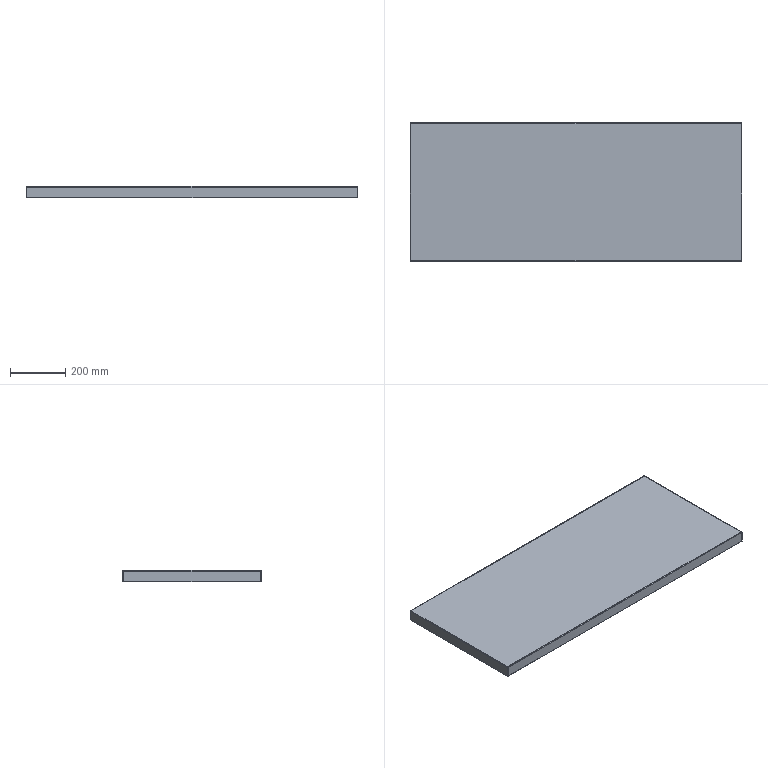Component | SolidWorks | CartChassis-1_BottomPlate-1 | 1 solid | 42 faces | box 1200 x 500 x 40.8 mm | volume 586293 mm3 | plane 34 | cylinder 8 | commonest cylinder face diameters 4.6 x4 3 x4 | material 304
STEP:
#1=COLOUR_RGB('',0.7922,0.8196,0.9333);
#2=FILL_AREA_STYLE_COLOUR('',#1);
#3=FILL_AREA_STYLE('',(#2));
#4=SURFACE_STYLE_FILL_AREA(#3);
#5=SURFACE_SIDE_STYLE('',(#4));
#6=SURFACE_STYLE_USAGE(.BOTH.,#5);
#7=PRESENTATION_STYLE_ASSIGNMENT((#6));
#8=CARTESIAN_POINT('',(-25.896,-8.479,48.12));
#9=VERTEX_POINT('',#8);
#10=CARTESIAN_POINT('',(-25.896,-8.457,48.12));
#11=VERTEX_POINT('',#10);
#12=CARTESIAN_POINT('',(-25.896,-8.479,48.12));
#13=DIRECTION('',(0.,1.,-0.));
#14=VECTOR('',#13,39.37);
#15=LINE('',#12,#14);
#16=EDGE_CURVE('',#9,#11,#15,.T.);
#17=ORIENTED_EDGE('',*,*,#16,.T.);
#18=CARTESIAN_POINT('',(-25.896,-8.389,48.152));
#19=VERTEX_POINT('',#18);
#20=CARTESIAN_POINT('',(-25.896,-8.389,48.061));
#21=DIRECTION('',(-1.,0.,0.));
#22=DIRECTION('',(0.,0.,-1.));
#23=AXIS2_PLACEMENT_3D('',#20,#21,#22);
#24=CIRCLE('',#23,0.09055);
#25=EDGE_CURVE('',#11,#19,#24,.T.);
#26=ORIENTED_EDGE('',*,*,#25,.T.);
#27=CARTESIAN_POINT('',(-25.896,-8.479,48.152));
#28=VERTEX_POINT('',#27);
#29=CARTESIAN_POINT('',(-25.896,11.206,48.152));
#30=DIRECTION('',(0.,1.,0.));
#31=VECTOR('',#30,39.37);
#32=LINE('',#29,#31);
#33=EDGE_CURVE('',#28,#19,#32,.T.);
#34=ORIENTED_EDGE('',*,*,#33,.F.);
#35=CARTESIAN_POINT('',(-25.896,-8.479,48.12));
#36=DIRECTION('',(0.,-0.,1.));
#37=VECTOR('',#36,39.37);
#38=LINE('',#35,#37);
#39=EDGE_CURVE('',#9,#28,#38,.T.);
#40=ORIENTED_EDGE('',*,*,#39,.F.);
#41=EDGE_LOOP('',(#17,#26,#34,#40));
#42=FACE_OUTER_BOUND('',#41,.T.);
#43=CARTESIAN_POINT('',(-25.896,-8.479,48.12));
#44=DIRECTION('',(1.,0.,-0.));
#45=DIRECTION('',(0.,-0.,1.));
#46=AXIS2_PLACEMENT_3D('',#43,#44,#45);
#47=PLANE('',#46);
#48=ADVANCED_FACE('',(#42),#47,.T.);
#49=CARTESIAN_POINT('',(21.167,-8.479,48.152));
#50=VERTEX_POINT('',#49);
#51=CARTESIAN_POINT('',(21.167,-8.389,48.152));
#52=VERTEX_POINT('',#51);
#53=CARTESIAN_POINT('',(21.167,-8.479,48.152));
#54=DIRECTION('',(0.,1.,0.));
#55=VECTOR('',#54,39.37);
#56=LINE('',#53,#55);
#57=EDGE_CURVE('',#50,#52,#56,.T.);
#58=ORIENTED_EDGE('',*,*,#57,.T.);
#59=CARTESIAN_POINT('',(21.167,-8.457,48.12));
#60=VERTEX_POINT('',#59);
#61=CARTESIAN_POINT('',(21.167,-8.389,48.061));
#62=DIRECTION('',(1.,-0.,-0.));
#63=DIRECTION('',(0.,-0.,-1.));
#64=AXIS2_PLACEMENT_3D('',#61,#62,#63);
#65=CIRCLE('',#64,0.09055);
#66=EDGE_CURVE('',#52,#60,#65,.T.);
#67=ORIENTED_EDGE('',*,*,#66,.T.);
#68=CARTESIAN_POINT('',(21.167,-8.479,48.12));
#69=VERTEX_POINT('',#68);
#70=CARTESIAN_POINT('',(21.167,-8.479,48.12));
#71=DIRECTION('',(0.,1.,0.));
#72=VECTOR('',#71,39.37);
#73=LINE('',#70,#72);
#74=EDGE_CURVE('',#69,#60,#73,.T.);
#75=ORIENTED_EDGE('',*,*,#74,.F.);
#76=CARTESIAN_POINT('',(21.167,-8.479,48.12));
#77=DIRECTION('',(0.,-0.,1.));
#78=VECTOR('',#77,39.37);
#79=LINE('',#76,#78);
#80=EDGE_CURVE('',#69,#50,#79,.T.);
#81=ORIENTED_EDGE('',*,*,#80,.T.);
#82=EDGE_LOOP('',(#58,#67,#75,#81));
#83=FACE_OUTER_BOUND('',#82,.T.);
#84=CARTESIAN_POINT('',(21.167,-8.389,48.12));
#85=DIRECTION('',(-1.,-0.,0.));
#86=DIRECTION('',(-0.,0.,-1.));
#87=AXIS2_PLACEMENT_3D('',#84,#85,#86);
#88=PLANE('',#87);
#89=ADVANCED_FACE('',(#83),#88,.T.);
#90=CARTESIAN_POINT('',(-25.896,11.115,48.152));
#91=VERTEX_POINT('',#90);
#92=CARTESIAN_POINT('',(-25.896,11.206,48.152));
#93=DIRECTION('',(-0.,-1.,-0.));
#94=VECTOR('',#93,39.37);
#95=LINE('',#92,#94);
#96=EDGE_CURVE('',#91,#19,#95,.T.);
#97=ORIENTED_EDGE('',*,*,#96,.T.);
#98=CARTESIAN_POINT('',(-25.896,-8.389,48.152));
#99=DIRECTION('',(1.,-0.,-0.));
#100=VECTOR('',#99,39.37);
#101=LINE('',#98,#100);
#102=EDGE_CURVE('',#19,#52,#101,.T.);
#103=ORIENTED_EDGE('',*,*,#102,.T.);
#104=CARTESIAN_POINT('',(21.167,11.115,48.152));
#105=VERTEX_POINT('',#104);
#106=CARTESIAN_POINT('',(21.167,-8.479,48.152));
#107=DIRECTION('',(0.,1.,0.));
#108=VECTOR('',#107,39.37);
#109=LINE('',#106,#108);
#110=EDGE_CURVE('',#52,#105,#109,.T.);
#111=ORIENTED_EDGE('',*,*,#110,.T.);
#112=CARTESIAN_POINT('',(21.167,11.115,48.152));
#113=DIRECTION('',(-1.,-0.,0.));
#114=VECTOR('',#113,39.37);
#115=LINE('',#112,#114);
#116=EDGE_CURVE('',#105,#91,#115,.T.);
#117=ORIENTED_EDGE('',*,*,#116,.T.);
#118=EDGE_LOOP('',(#97,#103,#111,#117));
#119=FACE_OUTER_BOUND('',#118,.T.);
#120=CARTESIAN_POINT('',(-2.365,1.363,48.152));
#121=DIRECTION('',(0.,-0.,1.));
#122=DIRECTION('',(-1.,-0.,0.));
#123=AXIS2_PLACEMENT_3D('',#120,#121,#122);
#124=PLANE('',#123);
#125=ADVANCED_FACE('',(#119),#124,.T.);
#126=CARTESIAN_POINT('',(-25.896,-8.389,48.12));
#127=VERTEX_POINT('',#126);
#128=CARTESIAN_POINT('',(21.167,-8.389,48.12));
#129=VERTEX_POINT('',#128);
#130=CARTESIAN_POINT('',(-25.896,-8.389,48.12));
#131=DIRECTION('',(1.,-0.,-0.));
#132=VECTOR('',#131,39.37);
#133=LINE('',#130,#132);
#134=EDGE_CURVE('',#127,#129,#133,.T.);
#135=ORIENTED_EDGE('',*,*,#134,.F.);
#136=CARTESIAN_POINT('',(-25.896,11.115,48.12));
#137=VERTEX_POINT('',#136);
#138=CARTESIAN_POINT('',(-25.896,11.206,48.12));
#139=DIRECTION('',(-0.,-1.,-0.));
#140=VECTOR('',#139,39.37);
#141=LINE('',#138,#140);
#142=EDGE_CURVE('',#137,#127,#141,.T.);
#143=ORIENTED_EDGE('',*,*,#142,.F.);
#144=CARTESIAN_POINT('',(21.167,11.115,48.12));
#145=VERTEX_POINT('',#144);
#146=CARTESIAN_POINT('',(21.167,11.115,48.12));
#147=DIRECTION('',(-1.,-0.,0.));
#148=VECTOR('',#147,39.37);
#149=LINE('',#146,#148);
#150=EDGE_CURVE('',#145,#137,#149,.T.);
#151=ORIENTED_EDGE('',*,*,#150,.F.);
#152=CARTESIAN_POINT('',(21.167,-8.479,48.12));
#153=DIRECTION('',(0.,1.,0.));
#154=VECTOR('',#153,39.37);
#155=LINE('',#152,#154);
#156=EDGE_CURVE('',#129,#145,#155,.T.);
#157=ORIENTED_EDGE('',*,*,#156,.F.);
#158=EDGE_LOOP('',(#135,#143,#151,#157));
#159=FACE_OUTER_BOUND('',#158,.T.);
#160=CARTESIAN_POINT('',(-2.365,1.363,48.12));
#161=DIRECTION('',(0.,-0.,1.));
#162=DIRECTION('',(-1.,-0.,0.));
#163=AXIS2_PLACEMENT_3D('',#160,#161,#162);
#164=PLANE('',#163);
#165=ADVANCED_FACE('',(#159),#164,.F.);
#166=CARTESIAN_POINT('',(21.167,11.206,48.12));
#167=VERTEX_POINT('',#166);
#168=CARTESIAN_POINT('',(21.167,11.184,48.12));
#169=VERTEX_POINT('',#168);
#170=CARTESIAN_POINT('',(21.167,11.206,48.12));
#171=DIRECTION('',(-0.,-1.,-0.));
#172=VECTOR('',#171,39.37);
#173=LINE('',#170,#172);
#174=EDGE_CURVE('',#167,#169,#173,.T.);
#175=ORIENTED_EDGE('',*,*,#174,.T.);
#176=CARTESIAN_POINT('',(21.167,11.115,48.061));
#177=DIRECTION('',(1.,0.,-0.));
#178=DIRECTION('',(0.,0.,1.));
#179=AXIS2_PLACEMENT_3D('',#176,#177,#178);
#180=CIRCLE('',#179,0.09055);
#181=EDGE_CURVE('',#169,#105,#180,.T.);
#182=ORIENTED_EDGE('',*,*,#181,.T.);
#183=CARTESIAN_POINT('',(21.167,11.206,48.152));
#184=VERTEX_POINT('',#183);
#185=CARTESIAN_POINT('',(21.167,-8.479,48.152));
#186=DIRECTION('',(-0.,-1.,-0.));
#187=VECTOR('',#186,39.37);
#188=LINE('',#185,#187);
#189=EDGE_CURVE('',#184,#105,#188,.T.);
#190=ORIENTED_EDGE('',*,*,#189,.F.);
#191=CARTESIAN_POINT('',(21.167,11.206,48.12));
#192=DIRECTION('',(0.,-0.,1.));
#193=VECTOR('',#192,39.37);
#194=LINE('',#191,#193);
#195=EDGE_CURVE('',#167,#184,#194,.T.);
#196=ORIENTED_EDGE('',*,*,#195,.F.);
#197=EDGE_LOOP('',(#175,#182,#190,#196));
#198=FACE_OUTER_BOUND('',#197,.T.);
#199=CARTESIAN_POINT('',(21.167,11.206,48.12));
#200=DIRECTION('',(-1.,-0.,0.));
#201=DIRECTION('',(-0.,0.,-1.));
#202=AXIS2_PLACEMENT_3D('',#199,#200,#201);
#203=PLANE('',#202);
#204=ADVANCED_FACE('',(#198),#203,.T.);
#205=CARTESIAN_POINT('',(-25.896,11.206,48.152));
#206=VERTEX_POINT('',#205);
#207=CARTESIAN_POINT('',(-25.896,11.206,48.152));
#208=DIRECTION('',(-0.,-1.,-0.));
#209=VECTOR('',#208,39.37);
#210=LINE('',#207,#209);
#211=EDGE_CURVE('',#206,#91,#210,.T.);
#212=ORIENTED_EDGE('',*,*,#211,.T.);
#213=CARTESIAN_POINT('',(-25.896,11.184,48.12));
#214=VERTEX_POINT('',#213);
#215=CARTESIAN_POINT('',(-25.896,11.115,48.061));
#216=DIRECTION('',(-1.,-0.,0.));
#217=DIRECTION('',(0.,0.,1.));
#218=AXIS2_PLACEMENT_3D('',#215,#216,#217);
#219=CIRCLE('',#218,0.09055);
#220=EDGE_CURVE('',#91,#214,#219,.T.);
#221=ORIENTED_EDGE('',*,*,#220,.T.);
#222=CARTESIAN_POINT('',(-25.896,11.206,48.12));
#223=VERTEX_POINT('',#222);
#224=CARTESIAN_POINT('',(-25.896,11.206,48.12));
#225=DIRECTION('',(-0.,-1.,-0.));
#226=VECTOR('',#225,39.37);
#227=LINE('',#224,#226);
#228=EDGE_CURVE('',#223,#214,#227,.T.);
#229=ORIENTED_EDGE('',*,*,#228,.F.);
#230=CARTESIAN_POINT('',(-25.896,11.206,48.12));
#231=DIRECTION('',(0.,-0.,1.));
#232=VECTOR('',#231,39.37);
#233=LINE('',#230,#232);
#234=EDGE_CURVE('',#223,#206,#233,.T.);
#235=ORIENTED_EDGE('',*,*,#234,.T.);
#236=EDGE_LOOP('',(#212,#221,#229,#235));
#237=FACE_OUTER_BOUND('',#236,.T.);
#238=CARTESIAN_POINT('',(-25.896,11.115,48.12));
#239=DIRECTION('',(1.,0.,-0.));
#240=DIRECTION('',(0.,-0.,1.));
#241=AXIS2_PLACEMENT_3D('',#238,#239,#240);
#242=PLANE('',#241);
#243=ADVANCED_FACE('',(#237),#242,.T.);
#244=CARTESIAN_POINT('',(21.226,11.206,48.061));
#245=VERTEX_POINT('',#244);
#246=CARTESIAN_POINT('',(21.257,11.206,48.061));
#247=VERTEX_POINT('',#246);
#248=CARTESIAN_POINT('',(21.257,11.206,48.061));
#249=DIRECTION('',(1.,-0.,0.));
#250=VECTOR('',#249,39.37);
#251=LINE('',#248,#250);
#252=EDGE_CURVE('',#245,#247,#251,.T.);
#253=ORIENTED_EDGE('',*,*,#252,.F.);
#254=CARTESIAN_POINT('',(21.167,11.206,48.061));
#255=DIRECTION('',(0.,1.,0.));
#256=DIRECTION('',(0.,0.,-1.));
#257=AXIS2_PLACEMENT_3D('',#254,#255,#256);
#258=CIRCLE('',#257,0.05906);
#259=EDGE_CURVE('',#167,#245,#258,.T.);
#260=ORIENTED_EDGE('',*,*,#259,.F.);
#261=ORIENTED_EDGE('',*,*,#195,.T.);
#262=CARTESIAN_POINT('',(21.167,11.206,48.061));
#263=DIRECTION('',(0.,1.,0.));
#264=DIRECTION('',(0.,0.,-1.));
#265=AXIS2_PLACEMENT_3D('',#262,#263,#264);
#266=CIRCLE('',#265,0.09055);
#267=EDGE_CURVE('',#184,#247,#266,.T.);
#268=ORIENTED_EDGE('',*,*,#267,.T.);
#269=EDGE_LOOP('',(#253,#260,#261,#268));
#270=FACE_OUTER_BOUND('',#269,.T.);
#271=CARTESIAN_POINT('',(21.167,11.206,48.061));
#272=DIRECTION('',(0.,1.,0.));
#273=DIRECTION('',(0.,-0.,1.));
#274=AXIS2_PLACEMENT_3D('',#271,#272,#273);
#275=PLANE('',#274);
#276=ADVANCED_FACE('',(#270),#275,.T.);
#277=CARTESIAN_POINT('',(21.226,-8.479,48.061));
#278=VERTEX_POINT('',#277);
#279=CARTESIAN_POINT('',(21.167,-8.479,48.061));
#280=DIRECTION('',(-0.,-1.,-0.));
#281=DIRECTION('',(0.,0.,-1.));
#282=AXIS2_PLACEMENT_3D('',#279,#280,#281);
#283=CIRCLE('',#282,0.05906);
#284=EDGE_CURVE('',#278,#69,#283,.T.);
#285=ORIENTED_EDGE('',*,*,#284,.F.);
#286=CARTESIAN_POINT('',(21.257,-8.479,48.061));
#287=VERTEX_POINT('',#286);
#288=CARTESIAN_POINT('',(21.226,-8.479,48.061));
#289=DIRECTION('',(1.,-0.,0.));
#290=VECTOR('',#289,39.37);
#291=LINE('',#288,#290);
#292=EDGE_CURVE('',#278,#287,#291,.T.);
#293=ORIENTED_EDGE('',*,*,#292,.T.);
#294=CARTESIAN_POINT('',(21.167,-8.479,48.061));
#295=DIRECTION('',(-0.,-1.,-0.));
#296=DIRECTION('',(0.,0.,-1.));
#297=AXIS2_PLACEMENT_3D('',#294,#295,#296);
#298=CIRCLE('',#297,0.09055);
#299=EDGE_CURVE('',#287,#50,#298,.T.);
#300=ORIENTED_EDGE('',*,*,#299,.T.);
#301=ORIENTED_EDGE('',*,*,#80,.F.);
#302=EDGE_LOOP('',(#285,#293,#300,#301));
#303=FACE_OUTER_BOUND('',#302,.T.);
#304=CARTESIAN_POINT('',(21.167,-8.479,48.061));
#305=DIRECTION('',(0.,1.,0.));
#306=DIRECTION('',(0.,-0.,1.));
#307=AXIS2_PLACEMENT_3D('',#304,#305,#306);
#308=PLANE('',#307);
#309=ADVANCED_FACE('',(#303),#308,.F.);
#310=ORIENTED_EDGE('',*,*,#57,.F.);
#311=ORIENTED_EDGE('',*,*,#299,.F.);
#312=CARTESIAN_POINT('',(21.257,1.363,48.061));
#313=DIRECTION('',(-0.,-1.,-0.));
#314=VECTOR('',#313,39.37);
#315=LINE('',#312,#314);
#316=EDGE_CURVE('',#247,#287,#315,.T.);
#317=ORIENTED_EDGE('',*,*,#316,.F.);
#318=ORIENTED_EDGE('',*,*,#267,.F.);
#319=ORIENTED_EDGE('',*,*,#189,.T.);
#320=ORIENTED_EDGE('',*,*,#110,.F.);
#321=EDGE_LOOP('',(#310,#311,#317,#318,#319,#320));
#322=FACE_OUTER_BOUND('',#321,.T.);
#323=CARTESIAN_POINT('',(21.167,-8.479,48.061));
#324=DIRECTION('',(-0.,-1.,-0.));
#325=DIRECTION('',(1.,0.,0.));
#326=AXIS2_PLACEMENT_3D('',#323,#324,#325);
#327=CYLINDRICAL_SURFACE('',#326,0.09055);
#328=ADVANCED_FACE('',(#322),#327,.T.);
#329=ORIENTED_EDGE('',*,*,#74,.T.);
#330=CARTESIAN_POINT('',(21.167,-8.479,48.12));
#331=DIRECTION('',(0.,1.,0.));
#332=VECTOR('',#331,39.37);
#333=LINE('',#330,#332);
#334=EDGE_CURVE('',#60,#129,#333,.T.);
#335=ORIENTED_EDGE('',*,*,#334,.T.);
#336=ORIENTED_EDGE('',*,*,#156,.T.);
#337=CARTESIAN_POINT('',(21.167,11.206,48.12));
#338=DIRECTION('',(-0.,-1.,-0.));
#339=VECTOR('',#338,39.37);
#340=LINE('',#337,#339);
#341=EDGE_CURVE('',#169,#145,#340,.T.);
#342=ORIENTED_EDGE('',*,*,#341,.F.);
#343=ORIENTED_EDGE('',*,*,#174,.F.);
#344=ORIENTED_EDGE('',*,*,#259,.T.);
#345=CARTESIAN_POINT('',(21.226,11.206,48.061));
#346=DIRECTION('',(-0.,-1.,-0.));
#347=VECTOR('',#346,39.37);
#348=LINE('',#345,#347);
#349=EDGE_CURVE('',#245,#278,#348,.T.);
#350=ORIENTED_EDGE('',*,*,#349,.T.);
#351=ORIENTED_EDGE('',*,*,#284,.T.);
#352=EDGE_LOOP('',(#329,#335,#336,#342,#343,#344,#350,#351));
#353=FACE_OUTER_BOUND('',#352,.T.);
#354=CARTESIAN_POINT('',(21.167,-8.479,48.061));
#355=DIRECTION('',(-0.,-1.,-0.));
#356=DIRECTION('',(1.,0.,0.));
#357=AXIS2_PLACEMENT_3D('',#354,#355,#356);
#358=CYLINDRICAL_SURFACE('',#357,0.05906);
#359=ADVANCED_FACE('',(#353),#358,.F.);
#360=CARTESIAN_POINT('',(21.257,-8.479,46.545));
#361=VERTEX_POINT('',#360);
#362=CARTESIAN_POINT('',(21.257,-8.479,48.12));
#363=DIRECTION('',(0.,-0.,1.));
#364=VECTOR('',#363,39.37);
#365=LINE('',#362,#364);
#366=EDGE_CURVE('',#361,#287,#365,.T.);
#367=ORIENTED_EDGE('',*,*,#366,.T.);
#368=ORIENTED_EDGE('',*,*,#292,.F.);
#369=CARTESIAN_POINT('',(21.226,-8.479,46.545));
#370=VERTEX_POINT('',#369);
#371=CARTESIAN_POINT('',(21.226,-8.479,48.12));
#372=DIRECTION('',(0.,-0.,1.));
#373=VECTOR('',#372,39.37);
#374=LINE('',#371,#373);
#375=EDGE_CURVE('',#370,#278,#374,.T.);
#376=ORIENTED_EDGE('',*,*,#375,.F.);
#377=CARTESIAN_POINT('',(21.257,-8.479,46.545));
#378=DIRECTION('',(-1.,0.,-0.));
#379=VECTOR('',#378,39.37);
#380=LINE('',#377,#379);
#381=EDGE_CURVE('',#361,#370,#380,.T.);
#382=ORIENTED_EDGE('',*,*,#381,.F.);
#383=EDGE_LOOP('',(#367,#368,#376,#382));
#384=FACE_OUTER_BOUND('',#383,.T.);
#385=CARTESIAN_POINT('',(21.257,-8.479,48.12));
#386=DIRECTION('',(-0.,-1.,-0.));
#387=DIRECTION('',(-0.,0.,-1.));
#388=AXIS2_PLACEMENT_3D('',#385,#386,#387);
#389=PLANE('',#388);
#390=ADVANCED_FACE('',(#384),#389,.T.);
#391=CARTESIAN_POINT('',(21.226,11.206,46.545));
#392=VERTEX_POINT('',#391);
#393=CARTESIAN_POINT('',(21.226,11.206,48.12));
#394=DIRECTION('',(-0.,0.,-1.));
#395=VECTOR('',#394,39.37);
#396=LINE('',#393,#395);
#397=EDGE_CURVE('',#245,#392,#396,.T.);
#398=ORIENTED_EDGE('',*,*,#397,.F.);
#399=ORIENTED_EDGE('',*,*,#252,.T.);
#400=CARTESIAN_POINT('',(21.257,11.206,46.545));
#401=VERTEX_POINT('',#400);
#402=CARTESIAN_POINT('',(21.257,11.206,46.545));
#403=DIRECTION('',(-0.,0.,-1.));
#404=VECTOR('',#403,39.37);
#405=LINE('',#402,#404);
#406=EDGE_CURVE('',#247,#401,#405,.T.);
#407=ORIENTED_EDGE('',*,*,#406,.T.);
#408=CARTESIAN_POINT('',(21.257,11.206,46.545));
#409=DIRECTION('',(-1.,0.,-0.));
#410=VECTOR('',#409,39.37);
#411=LINE('',#408,#410);
#412=EDGE_CURVE('',#401,#392,#411,.T.);
#413=ORIENTED_EDGE('',*,*,#412,.T.);
#414=EDGE_LOOP('',(#398,#399,#407,#413));
#415=FACE_OUTER_BOUND('',#414,.T.);
#416=CARTESIAN_POINT('',(21.257,11.206,46.545));
#417=DIRECTION('',(0.,1.,0.));
#418=DIRECTION('',(0.,-0.,1.));
#419=AXIS2_PLACEMENT_3D('',#416,#417,#418);
#420=PLANE('',#419);
#421=ADVANCED_FACE('',(#415),#420,.T.);
#422=ORIENTED_EDGE('',*,*,#406,.F.);
#423=ORIENTED_EDGE('',*,*,#316,.T.);
#424=ORIENTED_EDGE('',*,*,#366,.F.);
#425=CARTESIAN_POINT('',(21.257,-8.479,46.545));
#426=DIRECTION('',(-0.,-1.,-0.));
#427=VECTOR('',#426,39.37);
#428=LINE('',#425,#427);
#429=EDGE_CURVE('',#401,#361,#428,.T.);
#430=ORIENTED_EDGE('',*,*,#429,.F.);
#431=EDGE_LOOP('',(#422,#423,#424,#430));
#432=FACE_OUTER_BOUND('',#431,.T.);
#433=CARTESIAN_POINT('',(21.257,1.363,48.12));
#434=DIRECTION('',(1.,-0.,-0.));
#435=DIRECTION('',(0.,-0.,1.));
#436=AXIS2_PLACEMENT_3D('',#433,#434,#435);
#437=PLANE('',#436);
#438=ADVANCED_FACE('',(#432),#437,.T.);
#439=ORIENTED_EDGE('',*,*,#349,.F.);
#440=ORIENTED_EDGE('',*,*,#397,.T.);
#441=CARTESIAN_POINT('',(21.226,1.363,46.545));
#442=DIRECTION('',(-0.,-1.,-0.));
#443=VECTOR('',#442,39.37);
#444=LINE('',#441,#443);
#445=EDGE_CURVE('',#392,#370,#444,.T.);
#446=ORIENTED_EDGE('',*,*,#445,.T.);
#447=ORIENTED_EDGE('',*,*,#375,.T.);
#448=EDGE_LOOP('',(#439,#440,#446,#447));
#449=FACE_OUTER_BOUND('',#448,.T.);
#450=CARTESIAN_POINT('',(21.226,1.363,48.12));
#451=DIRECTION('',(1.,-0.,-0.));
#452=DIRECTION('',(0.,-0.,1.));
#453=AXIS2_PLACEMENT_3D('',#450,#451,#452);
#454=PLANE('',#453);
#455=ADVANCED_FACE('',(#449),#454,.F.);
#456=ORIENTED_EDGE('',*,*,#445,.F.);
#457=ORIENTED_EDGE('',*,*,#412,.F.);
#458=ORIENTED_EDGE('',*,*,#429,.T.);
#459=ORIENTED_EDGE('',*,*,#381,.T.);
#460=EDGE_LOOP('',(#456,#457,#458,#459));
#461=FACE_OUTER_BOUND('',#460,.T.);
#462=CARTESIAN_POINT('',(21.257,-8.479,46.545));
#463=DIRECTION('',(0.,0.,-1.));
#464=DIRECTION('',(1.,-0.,0.));
#465=AXIS2_PLACEMENT_3D('',#462,#463,#464);
#466=PLANE('',#465);
#467=ADVANCED_FACE('',(#461),#466,.T.);
#468=CARTESIAN_POINT('',(-25.955,-8.479,48.061));
#469=VERTEX_POINT('',#468);
#470=CARTESIAN_POINT('',(-25.987,-8.479,48.061));
#471=VERTEX_POINT('',#470);
#472=CARTESIAN_POINT('',(-25.987,-8.479,48.061));
#473=DIRECTION('',(-1.,-0.,0.));
#474=VECTOR('',#473,39.37);
#475=LINE('',#472,#474);
#476=EDGE_CURVE('',#469,#471,#475,.T.);
#477=ORIENTED_EDGE('',*,*,#476,.F.);
#478=CARTESIAN_POINT('',(-25.896,-8.479,48.061));
#479=DIRECTION('',(-0.,-1.,-0.));
#480=DIRECTION('',(0.,0.,1.));
#481=AXIS2_PLACEMENT_3D('',#478,#479,#480);
#482=CIRCLE('',#481,0.05906);
#483=EDGE_CURVE('',#9,#469,#482,.T.);
#484=ORIENTED_EDGE('',*,*,#483,.F.);
#485=ORIENTED_EDGE('',*,*,#39,.T.);
#486=CARTESIAN_POINT('',(-25.896,-8.479,48.061));
#487=DIRECTION('',(-0.,-1.,-0.));
#488=DIRECTION('',(0.,0.,1.));
#489=AXIS2_PLACEMENT_3D('',#486,#487,#488);
#490=CIRCLE('',#489,0.09055);
#491=EDGE_CURVE('',#28,#471,#490,.T.);
#492=ORIENTED_EDGE('',*,*,#491,.T.);
#493=EDGE_LOOP('',(#477,#484,#485,#492));
#494=FACE_OUTER_BOUND('',#493,.T.);
#495=CARTESIAN_POINT('',(-25.896,-8.479,48.061));
#496=DIRECTION('',(-0.,-1.,-0.));
#497=DIRECTION('',(-0.,0.,-1.));
#498=AXIS2_PLACEMENT_3D('',#495,#496,#497);
#499=PLANE('',#498);
#500=ADVANCED_FACE('',(#494),#499,.T.);
#501=CARTESIAN_POINT('',(-25.955,11.206,48.061));
#502=VERTEX_POINT('',#501);
#503=CARTESIAN_POINT('',(-25.896,11.206,48.061));
#504=DIRECTION('',(0.,1.,0.));
#505=DIRECTION('',(0.,0.,1.));
#506=AXIS2_PLACEMENT_3D('',#503,#504,#505);
#507=CIRCLE('',#506,0.05906);
#508=EDGE_CURVE('',#502,#223,#507,.T.);
#509=ORIENTED_EDGE('',*,*,#508,.F.);
#510=CARTESIAN_POINT('',(-25.987,11.206,48.061));
#511=VERTEX_POINT('',#510);
#512=CARTESIAN_POINT('',(-25.955,11.206,48.061));
#513=DIRECTION('',(-1.,-0.,0.));
#514=VECTOR('',#513,39.37);
#515=LINE('',#512,#514);
#516=EDGE_CURVE('',#502,#511,#515,.T.);
#517=ORIENTED_EDGE('',*,*,#516,.T.);
#518=CARTESIAN_POINT('',(-25.896,11.206,48.061));
#519=DIRECTION('',(0.,1.,0.));
#520=DIRECTION('',(0.,0.,1.));
#521=AXIS2_PLACEMENT_3D('',#518,#519,#520);
#522=CIRCLE('',#521,0.09055);
#523=EDGE_CURVE('',#511,#206,#522,.T.);
#524=ORIENTED_EDGE('',*,*,#523,.T.);
#525=ORIENTED_EDGE('',*,*,#234,.F.);
#526=EDGE_LOOP('',(#509,#517,#524,#525));
#527=FACE_OUTER_BOUND('',#526,.T.);
#528=CARTESIAN_POINT('',(-25.896,11.206,48.061));
#529=DIRECTION('',(-0.,-1.,-0.));
#530=DIRECTION('',(-0.,0.,-1.));
#531=AXIS2_PLACEMENT_3D('',#528,#529,#530);
#532=PLANE('',#531);
#533=ADVANCED_FACE('',(#527),#532,.F.);
#534=ORIENTED_EDGE('',*,*,#211,.F.);
#535=ORIENTED_EDGE('',*,*,#523,.F.);
#536=CARTESIAN_POINT('',(-25.987,-8.479,48.061));
#537=DIRECTION('',(-0.,-1.,-0.));
#538=VECTOR('',#537,39.37);
#539=LINE('',#536,#538);
#540=EDGE_CURVE('',#511,#471,#539,.T.);
#541=ORIENTED_EDGE('',*,*,#540,.T.);
#542=ORIENTED_EDGE('',*,*,#491,.F.);
#543=ORIENTED_EDGE('',*,*,#33,.T.);
#544=ORIENTED_EDGE('',*,*,#96,.F.);
#545=EDGE_LOOP('',(#534,#535,#541,#542,#543,#544));
#546=FACE_OUTER_BOUND('',#545,.T.);
#547=CARTESIAN_POINT('',(-25.896,11.206,48.061));
#548=DIRECTION('',(0.,1.,0.));
#549=DIRECTION('',(-1.,0.,0.));
#550=AXIS2_PLACEMENT_3D('',#547,#548,#549);
#551=CYLINDRICAL_SURFACE('',#550,0.09055);
#552=ADVANCED_FACE('',(#546),#551,.T.);
#553=ORIENTED_EDGE('',*,*,#228,.T.);
#554=CARTESIAN_POINT('',(-25.896,11.206,48.12));
#555=DIRECTION('',(-0.,-1.,-0.));
#556=VECTOR('',#555,39.37);
#557=LINE('',#554,#556);
#558=EDGE_CURVE('',#214,#137,#557,.T.);
#559=ORIENTED_EDGE('',*,*,#558,.T.);
#560=ORIENTED_EDGE('',*,*,#142,.T.);
#561=CARTESIAN_POINT('',(-25.896,-8.479,48.12));
#562=DIRECTION('',(0.,1.,-0.));
#563=VECTOR('',#562,39.37);
#564=LINE('',#561,#563);
#565=EDGE_CURVE('',#11,#127,#564,.T.);
#566=ORIENTED_EDGE('',*,*,#565,.F.);
#567=ORIENTED_EDGE('',*,*,#16,.F.);
#568=ORIENTED_EDGE('',*,*,#483,.T.);
#569=CARTESIAN_POINT('',(-25.955,-8.479,48.061));
#570=DIRECTION('',(0.,1.,0.));
#571=VECTOR('',#570,39.37);
#572=LINE('',#569,#571);
#573=EDGE_CURVE('',#469,#502,#572,.T.);
#574=ORIENTED_EDGE('',*,*,#573,.T.);
#575=ORIENTED_EDGE('',*,*,#508,.T.);
#576=EDGE_LOOP('',(#553,#559,#560,#566,#567,#568,#574,#575));
#577=FACE_OUTER_BOUND('',#576,.T.);
#578=CARTESIAN_POINT('',(-25.896,11.206,48.061));
#579=DIRECTION('',(0.,1.,0.));
#580=DIRECTION('',(-1.,0.,0.));
#581=AXIS2_PLACEMENT_3D('',#578,#579,#580);
#582=CYLINDRICAL_SURFACE('',#581,0.05906);
#583=ADVANCED_FACE('',(#577),#582,.F.);
#584=ORIENTED_EDGE('',*,*,#476,.T.);
#585=CARTESIAN_POINT('',(-25.987,-8.479,46.545));
#586=VERTEX_POINT('',#585);
#587=CARTESIAN_POINT('',(-25.987,-8.479,48.12));
#588=DIRECTION('',(0.,-0.,1.));
#589=VECTOR('',#588,39.37);
#590=LINE('',#587,#589);
#591=EDGE_CURVE('',#586,#471,#590,.T.);
#592=ORIENTED_EDGE('',*,*,#591,.F.);
#593=CARTESIAN_POINT('',(-25.955,-8.479,46.545));
#594=VERTEX_POINT('',#593);
#595=CARTESIAN_POINT('',(-25.987,-8.479,46.545));
#596=DIRECTION('',(1.,0.,-0.));
#597=VECTOR('',#596,39.37);
#598=LINE('',#595,#597);
#599=EDGE_CURVE('',#586,#594,#598,.T.);
#600=ORIENTED_EDGE('',*,*,#599,.T.);
#601=CARTESIAN_POINT('',(-25.955,-8.479,48.12));
#602=DIRECTION('',(0.,-0.,1.));
#603=VECTOR('',#602,39.37);
#604=LINE('',#601,#603);
#605=EDGE_CURVE('',#594,#469,#604,.T.);
#606=ORIENTED_EDGE('',*,*,#605,.T.);
#607=EDGE_LOOP('',(#584,#592,#600,#606));
#608=FACE_OUTER_BOUND('',#607,.T.);
#609=CARTESIAN_POINT('',(-25.987,-8.479,48.12));
#610=DIRECTION('',(0.,1.,0.));
#611=DIRECTION('',(0.,-0.,1.));
#612=AXIS2_PLACEMENT_3D('',#609,#610,#611);
#613=PLANE('',#612);
#614=ADVANCED_FACE('',(#608),#613,.F.);
#615=ORIENTED_EDGE('',*,*,#516,.F.);
#616=CARTESIAN_POINT('',(-25.955,11.206,46.545));
#617=VERTEX_POINT('',#616);
#618=CARTESIAN_POINT('',(-25.955,11.206,46.545));
#619=DIRECTION('',(-0.,0.,-1.));
#620=VECTOR('',#619,39.37);
#621=LINE('',#618,#620);
#622=EDGE_CURVE('',#502,#617,#621,.T.);
#623=ORIENTED_EDGE('',*,*,#622,.T.);
#624=CARTESIAN_POINT('',(-25.987,11.206,46.545));
#625=VERTEX_POINT('',#624);
#626=CARTESIAN_POINT('',(-25.987,11.206,46.545));
#627=DIRECTION('',(1.,0.,-0.));
#628=VECTOR('',#627,39.37);
#629=LINE('',#626,#628);
#630=EDGE_CURVE('',#625,#617,#629,.T.);
#631=ORIENTED_EDGE('',*,*,#630,.F.);
#632=CARTESIAN_POINT('',(-25.987,11.206,48.12));
#633=DIRECTION('',(-0.,0.,-1.));
#634=VECTOR('',#633,39.37);
#635=LINE('',#632,#634);
#636=EDGE_CURVE('',#511,#625,#635,.T.);
#637=ORIENTED_EDGE('',*,*,#636,.F.);
#638=EDGE_LOOP('',(#615,#623,#631,#637));
#639=FACE_OUTER_BOUND('',#638,.T.);
#640=CARTESIAN_POINT('',(-25.987,11.206,46.545));
#641=DIRECTION('',(-0.,-1.,-0.));
#642=DIRECTION('',(-0.,0.,-1.));
#643=AXIS2_PLACEMENT_3D('',#640,#641,#642);
#644=PLANE('',#643);
#645=ADVANCED_FACE('',(#639),#644,.F.);
#646=ORIENTED_EDGE('',*,*,#540,.F.);
#647=ORIENTED_EDGE('',*,*,#636,.T.);
#648=CARTESIAN_POINT('',(-25.987,1.363,46.545));
#649=DIRECTION('',(-0.,-1.,-0.));
#650=VECTOR('',#649,39.37);
#651=LINE('',#648,#650);
#652=EDGE_CURVE('',#625,#586,#651,.T.);
#653=ORIENTED_EDGE('',*,*,#652,.T.);
#654=ORIENTED_EDGE('',*,*,#591,.T.);
#655=EDGE_LOOP('',(#646,#647,#653,#654));
#656=FACE_OUTER_BOUND('',#655,.T.);
#657=CARTESIAN_POINT('',(-25.987,1.363,48.12));
#658=DIRECTION('',(1.,0.,-0.));
#659=DIRECTION('',(0.,-0.,1.));
#660=AXIS2_PLACEMENT_3D('',#657,#658,#659);
#661=PLANE('',#660);
#662=ADVANCED_FACE('',(#656),#661,.F.);
#663=ORIENTED_EDGE('',*,*,#622,.F.);
#664=ORIENTED_EDGE('',*,*,#573,.F.);
#665=ORIENTED_EDGE('',*,*,#605,.F.);
#666=CARTESIAN_POINT('',(-25.955,-8.479,46.545));
#667=DIRECTION('',(-0.,-1.,-0.));
#668=VECTOR('',#667,39.37);
#669=LINE('',#666,#668);
#670=EDGE_CURVE('',#617,#594,#669,.T.);
#671=ORIENTED_EDGE('',*,*,#670,.F.);
#672=EDGE_LOOP('',(#663,#664,#665,#671));
#673=FACE_OUTER_BOUND('',#672,.T.);
#674=CARTESIAN_POINT('',(-25.955,1.363,48.12));
#675=DIRECTION('',(1.,0.,-0.));
#676=DIRECTION('',(0.,-0.,1.));
#677=AXIS2_PLACEMENT_3D('',#674,#675,#676);
#678=PLANE('',#677);
#679=ADVANCED_FACE('',(#673),#678,.T.);
#680=ORIENTED_EDGE('',*,*,#670,.T.);
#681=ORIENTED_EDGE('',*,*,#599,.F.);
#682=ORIENTED_EDGE('',*,*,#652,.F.);
#683=ORIENTED_EDGE('',*,*,#630,.T.);
#684=EDGE_LOOP('',(#680,#681,#682,#683));
#685=FACE_OUTER_BOUND('',#684,.T.);
#686=CARTESIAN_POINT('',(-25.987,-8.479,46.545));
#687=DIRECTION('',(0.,-0.,1.));
#688=DIRECTION('',(-1.,-0.,0.));
#689=AXIS2_PLACEMENT_3D('',#686,#687,#688);
#690=PLANE('',#689);
#691=ADVANCED_FACE('',(#685),#690,.F.);
#692=ORIENTED_EDGE('',*,*,#558,.F.);
#693=CARTESIAN_POINT('',(-25.896,11.206,48.061));
#694=VERTEX_POINT('',#693);
#695=CARTESIAN_POINT('',(-25.896,11.115,48.061));
#696=DIRECTION('',(-1.,-0.,0.));
#697=DIRECTION('',(0.,0.,1.));
#698=AXIS2_PLACEMENT_3D('',#695,#696,#697);
#699=CIRCLE('',#698,0.09055);
#700=EDGE_CURVE('',#214,#694,#699,.T.);
#701=ORIENTED_EDGE('',*,*,#700,.T.);
#702=CARTESIAN_POINT('',(-25.896,11.174,48.061));
#703=VERTEX_POINT('',#702);
#704=CARTESIAN_POINT('',(-25.896,11.206,48.061));
#705=DIRECTION('',(0.,1.,0.));
#706=VECTOR('',#705,39.37);
#707=LINE('',#704,#706);
#708=EDGE_CURVE('',#703,#694,#707,.T.);
#709=ORIENTED_EDGE('',*,*,#708,.F.);
#710=CARTESIAN_POINT('',(-25.896,11.115,48.061));
#711=DIRECTION('',(-1.,-0.,0.));
#712=DIRECTION('',(0.,0.,1.));
#713=AXIS2_PLACEMENT_3D('',#710,#711,#712);
#714=CIRCLE('',#713,0.05906);
#715=EDGE_CURVE('',#137,#703,#714,.T.);
#716=ORIENTED_EDGE('',*,*,#715,.F.);
#717=EDGE_LOOP('',(#692,#701,#709,#716));
#718=FACE_OUTER_BOUND('',#717,.T.);
#719=CARTESIAN_POINT('',(-25.896,11.115,48.061));
#720=DIRECTION('',(-1.,-0.,0.));
#721=DIRECTION('',(-0.,0.,-1.));
#722=AXIS2_PLACEMENT_3D('',#719,#720,#721);
#723=PLANE('',#722);
#724=ADVANCED_FACE('',(#718),#723,.T.);
#725=CARTESIAN_POINT('',(21.167,11.206,48.061));
#726=VERTEX_POINT('',#725);
#727=CARTESIAN_POINT('',(21.167,11.115,48.061));
#728=DIRECTION('',(1.,0.,-0.));
#729=DIRECTION('',(0.,0.,1.));
#730=AXIS2_PLACEMENT_3D('',#727,#728,#729);
#731=CIRCLE('',#730,0.09055);
#732=EDGE_CURVE('',#726,#169,#731,.T.);
#733=ORIENTED_EDGE('',*,*,#732,.T.);
#734=ORIENTED_EDGE('',*,*,#341,.T.);
#735=CARTESIAN_POINT('',(21.167,11.174,48.061));
#736=VERTEX_POINT('',#735);
#737=CARTESIAN_POINT('',(21.167,11.115,48.061));
#738=DIRECTION('',(1.,0.,-0.));
#739=DIRECTION('',(0.,0.,1.));
#740=AXIS2_PLACEMENT_3D('',#737,#738,#739);
#741=CIRCLE('',#740,0.05906);
#742=EDGE_CURVE('',#736,#145,#741,.T.);
#743=ORIENTED_EDGE('',*,*,#742,.F.);
#744=CARTESIAN_POINT('',(21.167,11.174,48.061));
#745=DIRECTION('',(0.,1.,0.));
#746=VECTOR('',#745,39.37);
#747=LINE('',#744,#746);
#748=EDGE_CURVE('',#736,#726,#747,.T.);
#749=ORIENTED_EDGE('',*,*,#748,.T.);
#750=EDGE_LOOP('',(#733,#734,#743,#749));
#751=FACE_OUTER_BOUND('',#750,.T.);
#752=CARTESIAN_POINT('',(21.167,11.115,48.061));
#753=DIRECTION('',(-1.,-0.,0.));
#754=DIRECTION('',(-0.,0.,-1.));
#755=AXIS2_PLACEMENT_3D('',#752,#753,#754);
#756=PLANE('',#755);
#757=ADVANCED_FACE('',(#751),#756,.F.);
#758=ORIENTED_EDGE('',*,*,#116,.F.);
#759=ORIENTED_EDGE('',*,*,#181,.F.);
#760=ORIENTED_EDGE('',*,*,#732,.F.);
#761=CARTESIAN_POINT('',(-25.896,11.206,48.061));
#762=DIRECTION('',(-1.,-0.,0.));
#763=VECTOR('',#762,39.37);
#764=LINE('',#761,#763);
#765=EDGE_CURVE('',#726,#694,#764,.T.);
#766=ORIENTED_EDGE('',*,*,#765,.T.);
#767=ORIENTED_EDGE('',*,*,#700,.F.);
#768=ORIENTED_EDGE('',*,*,#220,.F.);
#769=EDGE_LOOP('',(#758,#759,#760,#766,#767,#768));
#770=FACE_OUTER_BOUND('',#769,.T.);
#771=CARTESIAN_POINT('',(21.167,11.115,48.061));
#772=DIRECTION('',(1.,0.,-0.));
#773=DIRECTION('',(0.,1.,0.));
#774=AXIS2_PLACEMENT_3D('',#771,#772,#773);
#775=CYLINDRICAL_SURFACE('',#774,0.09055);
#776=ADVANCED_FACE('',(#770),#775,.T.);
#777=ORIENTED_EDGE('',*,*,#150,.T.);
#778=ORIENTED_EDGE('',*,*,#715,.T.);
#779=CARTESIAN_POINT('',(-25.896,11.174,48.061));
#780=DIRECTION('',(1.,0.,-0.));
#781=VECTOR('',#780,39.37);
#782=LINE('',#779,#781);
#783=EDGE_CURVE('',#703,#736,#782,.T.);
#784=ORIENTED_EDGE('',*,*,#783,.T.);
#785=ORIENTED_EDGE('',*,*,#742,.T.);
#786=EDGE_LOOP('',(#777,#778,#784,#785));
#787=FACE_OUTER_BOUND('',#786,.T.);
#788=CARTESIAN_POINT('',(21.167,11.115,48.061));
#789=DIRECTION('',(1.,0.,-0.));
#790=DIRECTION('',(0.,1.,0.));
#791=AXIS2_PLACEMENT_3D('',#788,#789,#790);
#792=CYLINDRICAL_SURFACE('',#791,0.05906);
#793=ADVANCED_FACE('',(#787),#792,.F.);
#794=ORIENTED_EDGE('',*,*,#748,.F.);
#795=CARTESIAN_POINT('',(21.167,11.174,46.545));
#796=VERTEX_POINT('',#795);
#797=CARTESIAN_POINT('',(21.167,11.174,46.545));
#798=DIRECTION('',(-0.,0.,-1.));
#799=VECTOR('',#798,39.37);
#800=LINE('',#797,#799);
#801=EDGE_CURVE('',#736,#796,#800,.T.);
#802=ORIENTED_EDGE('',*,*,#801,.T.);
#803=CARTESIAN_POINT('',(21.167,11.206,46.545));
#804=VERTEX_POINT('',#803);
#805=CARTESIAN_POINT('',(21.167,11.206,46.545));
#806=DIRECTION('',(-0.,-1.,-0.));
#807=VECTOR('',#806,39.37);
#808=LINE('',#805,#807);
#809=EDGE_CURVE('',#804,#796,#808,.T.);
#810=ORIENTED_EDGE('',*,*,#809,.F.);
#811=CARTESIAN_POINT('',(21.167,11.206,48.12));
#812=DIRECTION('',(-0.,0.,-1.));
#813=VECTOR('',#812,39.37);
#814=LINE('',#811,#813);
#815=EDGE_CURVE('',#726,#804,#814,.T.);
#816=ORIENTED_EDGE('',*,*,#815,.F.);
#817=EDGE_LOOP('',(#794,#802,#810,#816));
#818=FACE_OUTER_BOUND('',#817,.T.);
#819=CARTESIAN_POINT('',(21.167,11.206,46.545));
#820=DIRECTION('',(-1.,-0.,0.));
#821=DIRECTION('',(-0.,0.,-1.));
#822=AXIS2_PLACEMENT_3D('',#819,#820,#821);
#823=PLANE('',#822);
#824=ADVANCED_FACE('',(#818),#823,.F.);
#825=ORIENTED_EDGE('',*,*,#708,.T.);
#826=CARTESIAN_POINT('',(-25.896,11.206,46.545));
#827=VERTEX_POINT('',#826);
#828=CARTESIAN_POINT('',(-25.896,11.206,48.12));
#829=DIRECTION('',(0.,-0.,1.));
#830=VECTOR('',#829,39.37);
#831=LINE('',#828,#830);
#832=EDGE_CURVE('',#827,#694,#831,.T.);
#833=ORIENTED_EDGE('',*,*,#832,.F.);
#834=CARTESIAN_POINT('',(-25.896,11.174,46.545));
#835=VERTEX_POINT('',#834);
#836=CARTESIAN_POINT('',(-25.896,11.206,46.545));
#837=DIRECTION('',(-0.,-1.,-0.));
#838=VECTOR('',#837,39.37);
#839=LINE('',#836,#838);
#840=EDGE_CURVE('',#827,#835,#839,.T.);
#841=ORIENTED_EDGE('',*,*,#840,.T.);
#842=CARTESIAN_POINT('',(-25.896,11.174,48.12));
#843=DIRECTION('',(0.,-0.,1.));
#844=VECTOR('',#843,39.37);
#845=LINE('',#842,#844);
#846=EDGE_CURVE('',#835,#703,#845,.T.);
#847=ORIENTED_EDGE('',*,*,#846,.T.);
#848=EDGE_LOOP('',(#825,#833,#841,#847));
#849=FACE_OUTER_BOUND('',#848,.T.);
#850=CARTESIAN_POINT('',(-25.896,11.206,48.12));
#851=DIRECTION('',(1.,0.,-0.));
#852=DIRECTION('',(0.,-0.,1.));
#853=AXIS2_PLACEMENT_3D('',#850,#851,#852);
#854=PLANE('',#853);
#855=ADVANCED_FACE('',(#849),#854,.F.);
#856=ORIENTED_EDGE('',*,*,#765,.F.);
#857=ORIENTED_EDGE('',*,*,#815,.T.);
#858=CARTESIAN_POINT('',(-2.365,11.206,46.545));
#859=DIRECTION('',(-1.,-0.,0.));
#860=VECTOR('',#859,39.37);
#861=LINE('',#858,#860);
#862=EDGE_CURVE('',#804,#827,#861,.T.);
#863=ORIENTED_EDGE('',*,*,#862,.T.);
#864=ORIENTED_EDGE('',*,*,#832,.T.);
#865=EDGE_LOOP('',(#856,#857,#863,#864));
#866=FACE_OUTER_BOUND('',#865,.T.);
#867=CARTESIAN_POINT('',(-2.365,11.206,48.12));
#868=DIRECTION('',(-0.,-1.,-0.));
#869=DIRECTION('',(-0.,0.,-1.));
#870=AXIS2_PLACEMENT_3D('',#867,#868,#869);
#871=PLANE('',#870);
#872=ADVANCED_FACE('',(#866),#871,.F.);
#873=ORIENTED_EDGE('',*,*,#801,.F.);
#874=ORIENTED_EDGE('',*,*,#783,.F.);
#875=ORIENTED_EDGE('',*,*,#846,.F.);
#876=CARTESIAN_POINT('',(-25.896,11.174,46.545));
#877=DIRECTION('',(-1.,-0.,0.));
#878=VECTOR('',#877,39.37);
#879=LINE('',#876,#878);
#880=EDGE_CURVE('',#796,#835,#879,.T.);
#881=ORIENTED_EDGE('',*,*,#880,.F.);
#882=EDGE_LOOP('',(#873,#874,#875,#881));
#883=FACE_OUTER_BOUND('',#882,.T.);
#884=CARTESIAN_POINT('',(-2.365,11.174,48.12));
#885=DIRECTION('',(-0.,-1.,-0.));
#886=DIRECTION('',(-0.,0.,-1.));
#887=AXIS2_PLACEMENT_3D('',#884,#885,#886);
#888=PLANE('',#887);
#889=ADVANCED_FACE('',(#883),#888,.T.);
#890=ORIENTED_EDGE('',*,*,#880,.T.);
#891=ORIENTED_EDGE('',*,*,#840,.F.);
#892=ORIENTED_EDGE('',*,*,#862,.F.);
#893=ORIENTED_EDGE('',*,*,#809,.T.);
#894=EDGE_LOOP('',(#890,#891,#892,#893));
#895=FACE_OUTER_BOUND('',#894,.T.);
#896=CARTESIAN_POINT('',(-25.896,11.206,46.545));
#897=DIRECTION('',(0.,-0.,1.));
#898=DIRECTION('',(-0.,-1.,-0.));
#899=AXIS2_PLACEMENT_3D('',#896,#897,#898);
#900=PLANE('',#899);
#901=ADVANCED_FACE('',(#895),#900,.F.);
#902=ORIENTED_EDGE('',*,*,#334,.F.);
#903=CARTESIAN_POINT('',(21.167,-8.479,48.061));
#904=VERTEX_POINT('',#903);
#905=CARTESIAN_POINT('',(21.167,-8.389,48.061));
#906=DIRECTION('',(1.,-0.,-0.));
#907=DIRECTION('',(0.,0.,-1.));
#908=AXIS2_PLACEMENT_3D('',#905,#906,#907);
#909=CIRCLE('',#908,0.09055);
#910=EDGE_CURVE('',#60,#904,#909,.T.);
#911=ORIENTED_EDGE('',*,*,#910,.T.);
#912=CARTESIAN_POINT('',(21.167,-8.448,48.061));
#913=VERTEX_POINT('',#912);
#914=CARTESIAN_POINT('',(21.167,-8.479,48.061));
#915=DIRECTION('',(-0.,-1.,-0.));
#916=VECTOR('',#915,39.37);
#917=LINE('',#914,#916);
#918=EDGE_CURVE('',#913,#904,#917,.T.);
#919=ORIENTED_EDGE('',*,*,#918,.F.);
#920=CARTESIAN_POINT('',(21.167,-8.389,48.061));
#921=DIRECTION('',(1.,-0.,-0.));
#922=DIRECTION('',(0.,0.,-1.));
#923=AXIS2_PLACEMENT_3D('',#920,#921,#922);
#924=CIRCLE('',#923,0.05906);
#925=EDGE_CURVE('',#129,#913,#924,.T.);
#926=ORIENTED_EDGE('',*,*,#925,.F.);
#927=EDGE_LOOP('',(#902,#911,#919,#926));
#928=FACE_OUTER_BOUND('',#927,.T.);
#929=CARTESIAN_POINT('',(21.167,-8.389,48.061));
#930=DIRECTION('',(1.,-0.,-0.));
#931=DIRECTION('',(0.,-0.,1.));
#932=AXIS2_PLACEMENT_3D('',#929,#930,#931);
#933=PLANE('',#932);
#934=ADVANCED_FACE('',(#928),#933,.T.);
#935=CARTESIAN_POINT('',(-25.896,-8.479,48.061));
#936=VERTEX_POINT('',#935);
#937=CARTESIAN_POINT('',(-25.896,-8.389,48.061));
#938=DIRECTION('',(-1.,0.,0.));
#939=DIRECTION('',(0.,0.,-1.));
#940=AXIS2_PLACEMENT_3D('',#937,#938,#939);
#941=CIRCLE('',#940,0.09055);
#942=EDGE_CURVE('',#936,#11,#941,.T.);
#943=ORIENTED_EDGE('',*,*,#942,.T.);
#944=ORIENTED_EDGE('',*,*,#565,.T.);
#945=CARTESIAN_POINT('',(-25.896,-8.448,48.061));
#946=VERTEX_POINT('',#945);
#947=CARTESIAN_POINT('',(-25.896,-8.389,48.061));
#948=DIRECTION('',(-1.,0.,0.));
#949=DIRECTION('',(0.,0.,-1.));
#950=AXIS2_PLACEMENT_3D('',#947,#948,#949);
#951=CIRCLE('',#950,0.05906);
#952=EDGE_CURVE('',#946,#127,#951,.T.);
#953=ORIENTED_EDGE('',*,*,#952,.F.);
#954=CARTESIAN_POINT('',(-25.896,-8.448,48.061));
#955=DIRECTION('',(-0.,-1.,-0.));
#956=VECTOR('',#955,39.37);
#957=LINE('',#954,#956);
#958=EDGE_CURVE('',#946,#936,#957,.T.);
#959=ORIENTED_EDGE('',*,*,#958,.T.);
#960=EDGE_LOOP('',(#943,#944,#953,#959));
#961=FACE_OUTER_BOUND('',#960,.T.);
#962=CARTESIAN_POINT('',(-25.896,-8.389,48.061));
#963=DIRECTION('',(1.,-0.,-0.));
#964=DIRECTION('',(0.,-0.,1.));
#965=AXIS2_PLACEMENT_3D('',#962,#963,#964);
#966=PLANE('',#965);
#967=ADVANCED_FACE('',(#961),#966,.F.);
#968=ORIENTED_EDGE('',*,*,#102,.F.);
#969=ORIENTED_EDGE('',*,*,#25,.F.);
#970=ORIENTED_EDGE('',*,*,#942,.F.);
#971=CARTESIAN_POINT('',(21.167,-8.479,48.061));
#972=DIRECTION('',(1.,0.,-0.));
#973=VECTOR('',#972,39.37);
#974=LINE('',#971,#973);
#975=EDGE_CURVE('',#936,#904,#974,.T.);
#976=ORIENTED_EDGE('',*,*,#975,.T.);
#977=ORIENTED_EDGE('',*,*,#910,.F.);
#978=ORIENTED_EDGE('',*,*,#66,.F.);
#979=EDGE_LOOP('',(#968,#969,#970,#976,#977,#978));
#980=FACE_OUTER_BOUND('',#979,.T.);
#981=CARTESIAN_POINT('',(-25.896,-8.389,48.061));
#982=DIRECTION('',(-1.,0.,0.));
#983=DIRECTION('',(0.,-1.,0.));
#984=AXIS2_PLACEMENT_3D('',#981,#982,#983);
#985=CYLINDRICAL_SURFACE('',#984,0.09055);
#986=ADVANCED_FACE('',(#980),#985,.T.);
#987=ORIENTED_EDGE('',*,*,#134,.T.);
#988=ORIENTED_EDGE('',*,*,#925,.T.);
#989=CARTESIAN_POINT('',(21.167,-8.448,48.061));
#990=DIRECTION('',(-1.,-0.,0.));
#991=VECTOR('',#990,39.37);
#992=LINE('',#989,#991);
#993=EDGE_CURVE('',#913,#946,#992,.T.);
#994=ORIENTED_EDGE('',*,*,#993,.T.);
#995=ORIENTED_EDGE('',*,*,#952,.T.);
#996=EDGE_LOOP('',(#987,#988,#994,#995));
#997=FACE_OUTER_BOUND('',#996,.T.);
#998=CARTESIAN_POINT('',(-25.896,-8.389,48.061));
#999=DIRECTION('',(-1.,0.,0.));
#1000=DIRECTION('',(0.,-1.,0.));
#1001=AXIS2_PLACEMENT_3D('',#998,#999,#1000);
#1002=CYLINDRICAL_SURFACE('',#1001,0.05906);
#1003=ADVANCED_FACE('',(#997),#1002,.F.);
#1004=ORIENTED_EDGE('',*,*,#918,.T.);
#1005=CARTESIAN_POINT('',(21.167,-8.479,46.545));
#1006=VERTEX_POINT('',#1005);
#1007=CARTESIAN_POINT('',(21.167,-8.479,48.12));
#1008=DIRECTION('',(0.,0.,1.));
#1009=VECTOR('',#1008,39.37);
#1010=LINE('',#1007,#1009);
#1011=EDGE_CURVE('',#1006,#904,#1010,.T.);
#1012=ORIENTED_EDGE('',*,*,#1011,.F.);
#1013=CARTESIAN_POINT('',(21.167,-8.448,46.545));
#1014=VERTEX_POINT('',#1013);
#1015=CARTESIAN_POINT('',(21.167,-8.479,46.545));
#1016=DIRECTION('',(0.,1.,0.));
#1017=VECTOR('',#1016,39.37);
#1018=LINE('',#1015,#1017);
#1019=EDGE_CURVE('',#1006,#1014,#1018,.T.);
#1020=ORIENTED_EDGE('',*,*,#1019,.T.);
#1021=CARTESIAN_POINT('',(21.167,-8.448,48.12));
#1022=DIRECTION('',(0.,0.,1.));
#1023=VECTOR('',#1022,39.37);
#1024=LINE('',#1021,#1023);
#1025=EDGE_CURVE('',#1014,#913,#1024,.T.);
#1026=ORIENTED_EDGE('',*,*,#1025,.T.);
#1027=EDGE_LOOP('',(#1004,#1012,#1020,#1026));
#1028=FACE_OUTER_BOUND('',#1027,.T.);
#1029=CARTESIAN_POINT('',(21.167,-8.479,48.12));
#1030=DIRECTION('',(-1.,-0.,0.));
#1031=DIRECTION('',(-0.,0.,-1.));
#1032=AXIS2_PLACEMENT_3D('',#1029,#1030,#1031);
#1033=PLANE('',#1032);
#1034=ADVANCED_FACE('',(#1028),#1033,.F.);
#1035=ORIENTED_EDGE('',*,*,#958,.F.);
#1036=CARTESIAN_POINT('',(-25.896,-8.448,46.545));
#1037=VERTEX_POINT('',#1036);
#1038=CARTESIAN_POINT('',(-25.896,-8.448,46.545));
#1039=DIRECTION('',(-0.,-0.,-1.));
#1040=VECTOR('',#1039,39.37);
#1041=LINE('',#1038,#1040);
#1042=EDGE_CURVE('',#946,#1037,#1041,.T.);
#1043=ORIENTED_EDGE('',*,*,#1042,.T.);
#1044=CARTESIAN_POINT('',(-25.896,-8.479,46.545));
#1045=VERTEX_POINT('',#1044);
#1046=CARTESIAN_POINT('',(-25.896,-8.479,46.545));
#1047=DIRECTION('',(0.,1.,0.));
#1048=VECTOR('',#1047,39.37);
#1049=LINE('',#1046,#1048);
#1050=EDGE_CURVE('',#1045,#1037,#1049,.T.);
#1051=ORIENTED_EDGE('',*,*,#1050,.F.);
#1052=CARTESIAN_POINT('',(-25.896,-8.479,48.12));
#1053=DIRECTION('',(-0.,-0.,-1.));
#1054=VECTOR('',#1053,39.37);
#1055=LINE('',#1052,#1054);
#1056=EDGE_CURVE('',#936,#1045,#1055,.T.);
#1057=ORIENTED_EDGE('',*,*,#1056,.F.);
#1058=EDGE_LOOP('',(#1035,#1043,#1051,#1057));
#1059=FACE_OUTER_BOUND('',#1058,.T.);
#1060=CARTESIAN_POINT('',(-25.896,-8.479,46.545));
#1061=DIRECTION('',(1.,0.,-0.));
#1062=DIRECTION('',(0.,-0.,1.));
#1063=AXIS2_PLACEMENT_3D('',#1060,#1061,#1062);
#1064=PLANE('',#1063);
#1065=ADVANCED_FACE('',(#1059),#1064,.F.);
#1066=ORIENTED_EDGE('',*,*,#975,.F.);
#1067=ORIENTED_EDGE('',*,*,#1056,.T.);
#1068=CARTESIAN_POINT('',(-2.365,-8.479,46.545));
#1069=DIRECTION('',(1.,0.,-0.));
#1070=VECTOR('',#1069,39.37);
#1071=LINE('',#1068,#1070);
#1072=EDGE_CURVE('',#1045,#1006,#1071,.T.);
#1073=ORIENTED_EDGE('',*,*,#1072,.T.);
#1074=ORIENTED_EDGE('',*,*,#1011,.T.);
#1075=EDGE_LOOP('',(#1066,#1067,#1073,#1074));
#1076=FACE_OUTER_BOUND('',#1075,.T.);
#1077=CARTESIAN_POINT('',(-2.365,-8.479,48.12));
#1078=DIRECTION('',(0.,1.,-0.));
#1079=DIRECTION('',(0.,0.,1.));
#1080=AXIS2_PLACEMENT_3D('',#1077,#1078,#1079);
#1081=PLANE('',#1080);
#1082=ADVANCED_FACE('',(#1076),#1081,.F.);
#1083=ORIENTED_EDGE('',*,*,#1042,.F.);
#1084=ORIENTED_EDGE('',*,*,#993,.F.);
#1085=ORIENTED_EDGE('',*,*,#1025,.F.);
#1086=CARTESIAN_POINT('',(21.167,-8.448,46.545));
#1087=DIRECTION('',(1.,0.,-0.));
#1088=VECTOR('',#1087,39.37);
#1089=LINE('',#1086,#1088);
#1090=EDGE_CURVE('',#1037,#1014,#1089,.T.);
#1091=ORIENTED_EDGE('',*,*,#1090,.F.);
#1092=EDGE_LOOP('',(#1083,#1084,#1085,#1091));
#1093=FACE_OUTER_BOUND('',#1092,.T.);
#1094=CARTESIAN_POINT('',(-2.365,-8.448,48.12));
#1095=DIRECTION('',(0.,1.,-0.));
#1096=DIRECTION('',(0.,0.,1.));
#1097=AXIS2_PLACEMENT_3D('',#1094,#1095,#1096);
#1098=PLANE('',#1097);
#1099=ADVANCED_FACE('',(#1093),#1098,.T.);
#1100=ORIENTED_EDGE('',*,*,#1090,.T.);
#1101=ORIENTED_EDGE('',*,*,#1019,.F.);
#1102=ORIENTED_EDGE('',*,*,#1072,.F.);
#1103=ORIENTED_EDGE('',*,*,#1050,.T.);
#1104=EDGE_LOOP('',(#1100,#1101,#1102,#1103));
#1105=FACE_OUTER_BOUND('',#1104,.T.);
#1106=CARTESIAN_POINT('',(21.167,-8.479,46.545));
#1107=DIRECTION('',(0.,-0.,1.));
#1108=DIRECTION('',(-0.,-1.,-0.));
#1109=AXIS2_PLACEMENT_3D('',#1106,#1107,#1108);
#1110=PLANE('',#1109);
#1111=ADVANCED_FACE('',(#1105),#1110,.F.);
#1112=CLOSED_SHELL('',(#48,#89,#125,#165,#204,#243,#276,#309,#328,#359,#390,#421,#438,#455,#467,#500,#533,#552,#583,#614,#645,#662,#679,#691,#724,#757,#776,#793,#824,#855,#872,#889,#901,#934,#967,#986,#1003,#1034,#1065,#1082,#1099,#1111));
#1113=MANIFOLD_SOLID_BREP('',#1112);
#1114=STYLED_ITEM('',(#7),#1113);
#1115=(LENGTH_UNIT()NAMED_UNIT(*)SI_UNIT($,.METRE.));
#1116=LENGTH_MEASURE_WITH_UNIT(LENGTH_MEASURE(0.0254),#1115);
#1117=DIMENSIONAL_EXPONENTS(1.,0.,0.,0.,0.,0.,0.);
#1118=(CONVERSION_BASED_UNIT('',#1116)LENGTH_UNIT()NAMED_UNIT(#1117));
#1119=UNCERTAINTY_MEASURE_WITH_UNIT(LENGTH_MEASURE(0.00001),#1118,'','');
#1120=(NAMED_UNIT(*)PLANE_ANGLE_UNIT()SI_UNIT($,.RADIAN.));
#1121=(NAMED_UNIT(*)SI_UNIT($,.STERADIAN.)SOLID_ANGLE_UNIT());
#1122=(GEOMETRIC_REPRESENTATION_CONTEXT(3)GLOBAL_UNCERTAINTY_ASSIGNED_CONTEXT((#1119))GLOBAL_UNIT_ASSIGNED_CONTEXT((#1118,#1120,#1121))REPRESENTATION_CONTEXT('',''));
#1123=MECHANICAL_DESIGN_GEOMETRIC_PRESENTATION_REPRESENTATION('',(#1114),#1122);
#1124=CARTESIAN_POINT('',(0.,0.,0.));
#1125=DIRECTION('',(0.,0.,1.));
#1126=DIRECTION('',(1.,0.,0.));
#1127=AXIS2_PLACEMENT_3D('',#1124,#1125,#1126);
#1128=(LENGTH_UNIT()NAMED_UNIT(*)SI_UNIT($,.METRE.));
#1129=LENGTH_MEASURE_WITH_UNIT(LENGTH_MEASURE(0.0254),#1128);
#1130=DIMENSIONAL_EXPONENTS(1.,0.,0.,0.,0.,0.,0.);
#1131=(CONVERSION_BASED_UNIT('',#1129)LENGTH_UNIT()NAMED_UNIT(#1130));
#1132=UNCERTAINTY_MEASURE_WITH_UNIT(LENGTH_MEASURE(0.00001),#1131,'','');
#1133=(NAMED_UNIT(*)PLANE_ANGLE_UNIT()SI_UNIT($,.RADIAN.));
#1134=(NAMED_UNIT(*)SI_UNIT($,.STERADIAN.)SOLID_ANGLE_UNIT());
#1135=(GEOMETRIC_REPRESENTATION_CONTEXT(3)GLOBAL_UNCERTAINTY_ASSIGNED_CONTEXT((#1132))GLOBAL_UNIT_ASSIGNED_CONTEXT((#1131,#1133,#1134))REPRESENTATION_CONTEXT('',''));
#1136=ADVANCED_BREP_SHAPE_REPRESENTATION('',(#1113,#1127),#1135);
#1137=PRESENTATION_LAYER_ASSIGNMENT('','',(#1114));